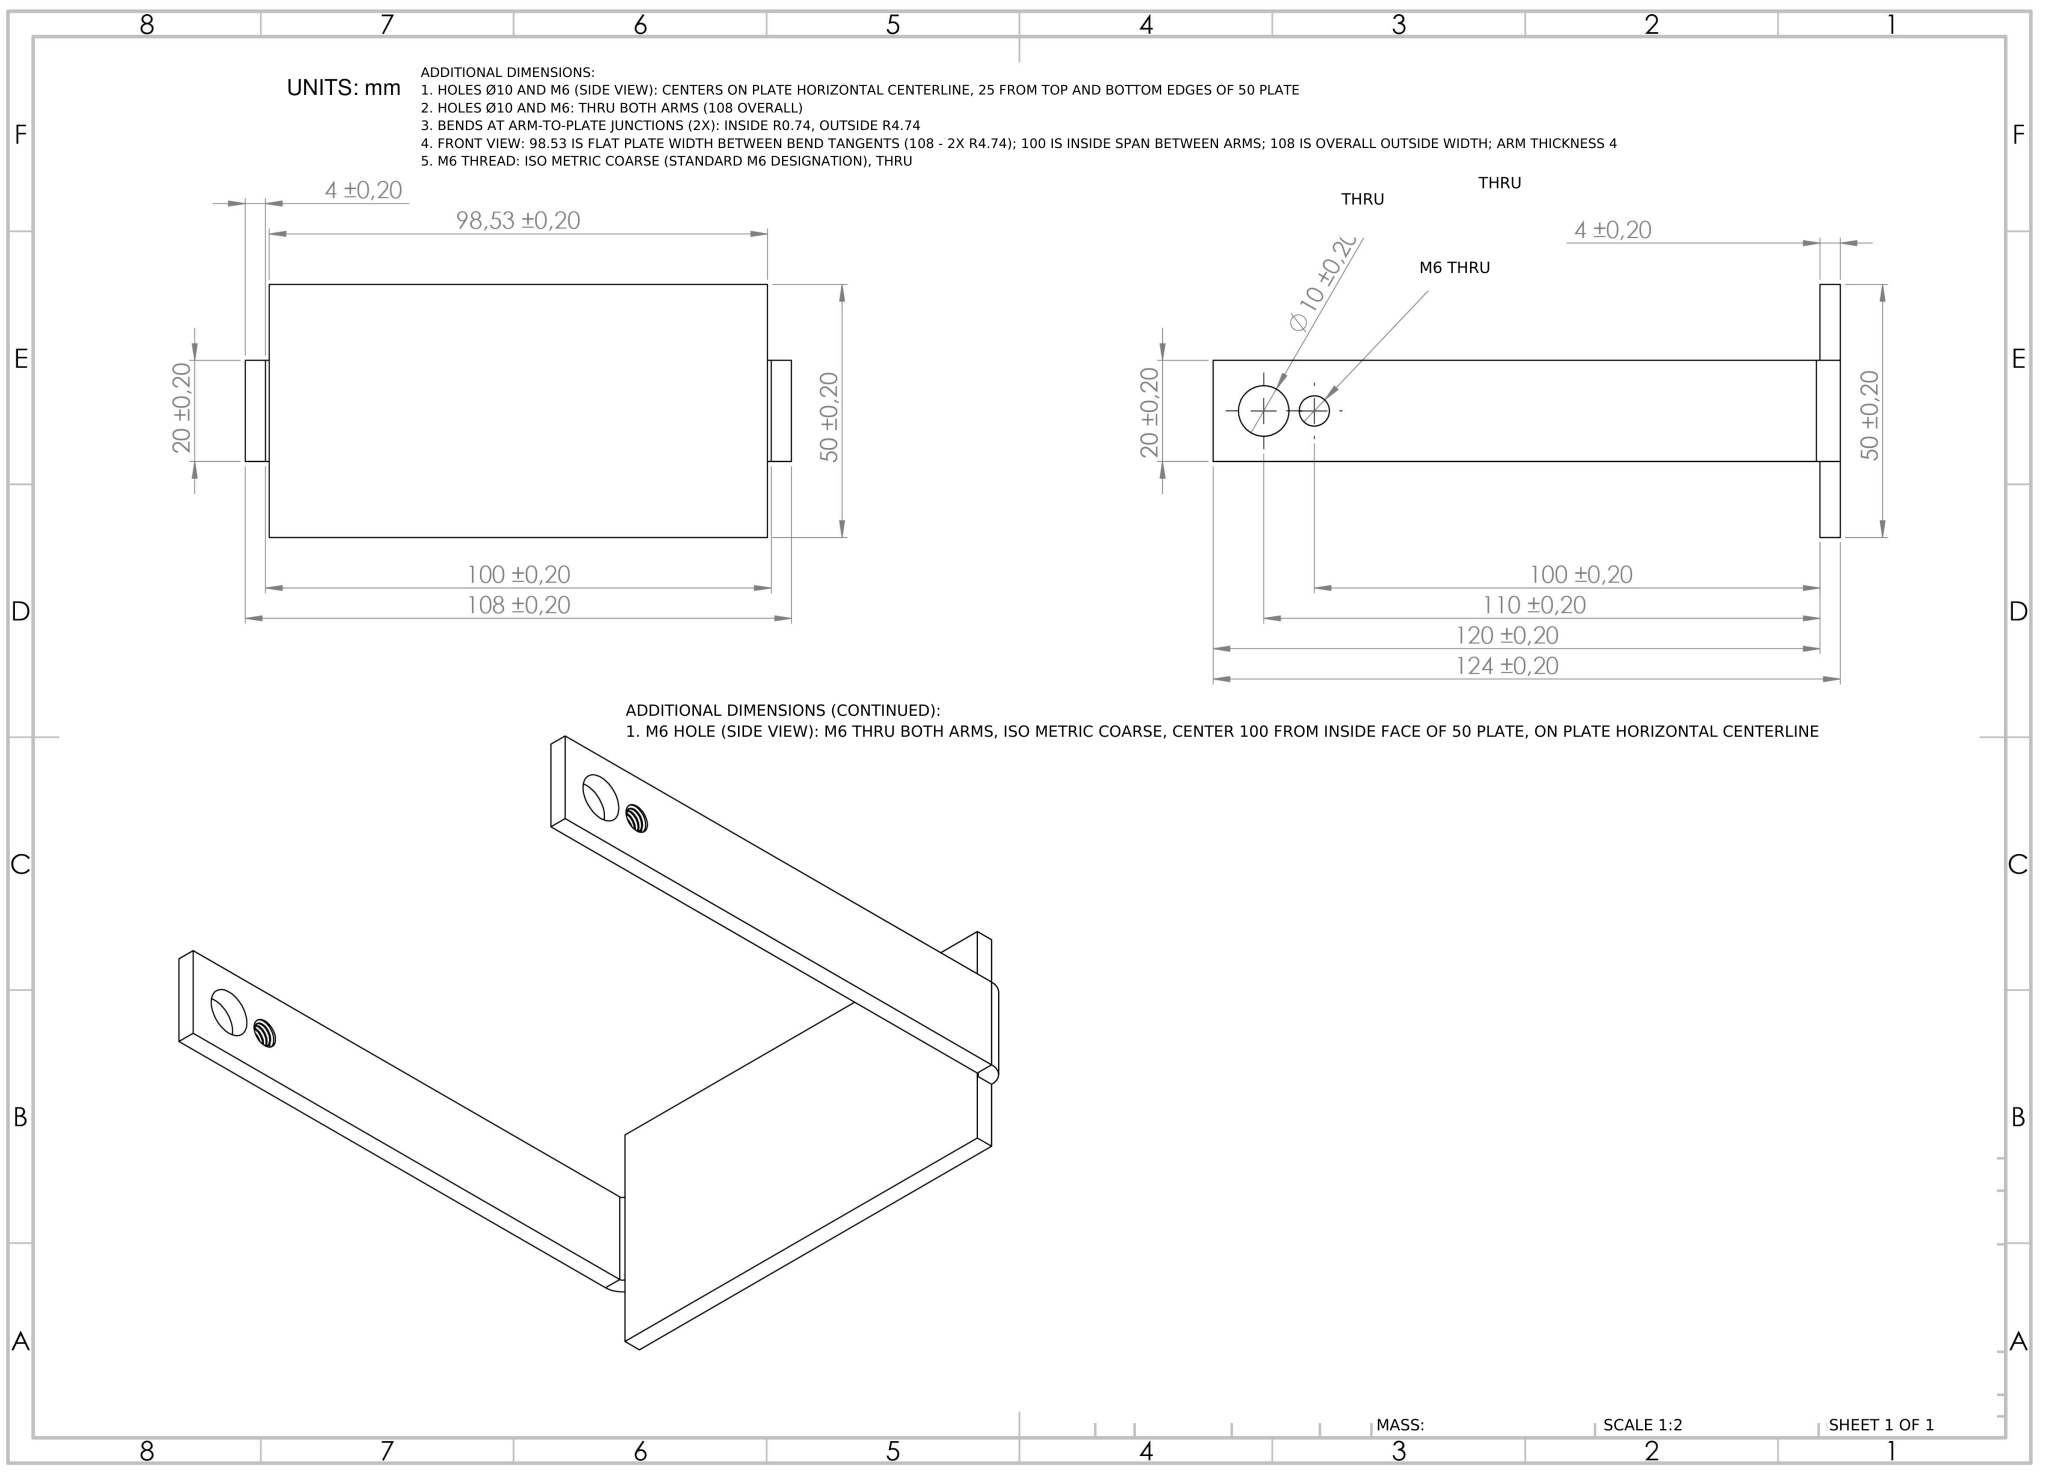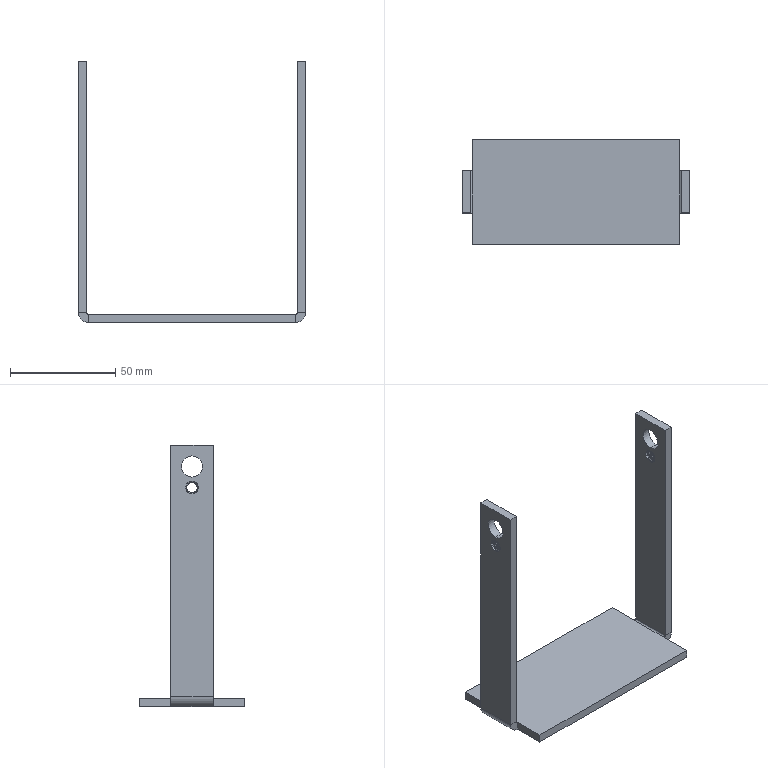Part | NX | mm | 1 solid | 61 faces | box 108 x 50 x 124 mm | volume 38655 mm3 | plane 31 | cylinder 24 | spline 6 | commonest cylinder face diameters 6 x16 10 x4 9.473 x2 1.473 x2